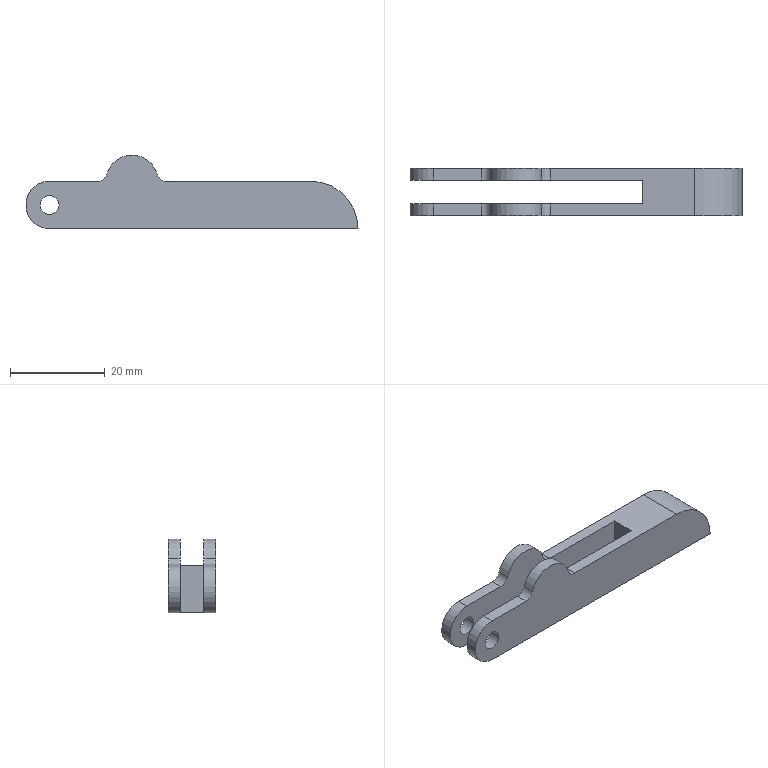Component | NX | RETAINER_PLATE | 1 solid | 20 faces | volume 4462 mm3 | cylinder 11 | plane 9 | commonest cylinder face diameters 4 x6 10 x2 11 x2 20 x1